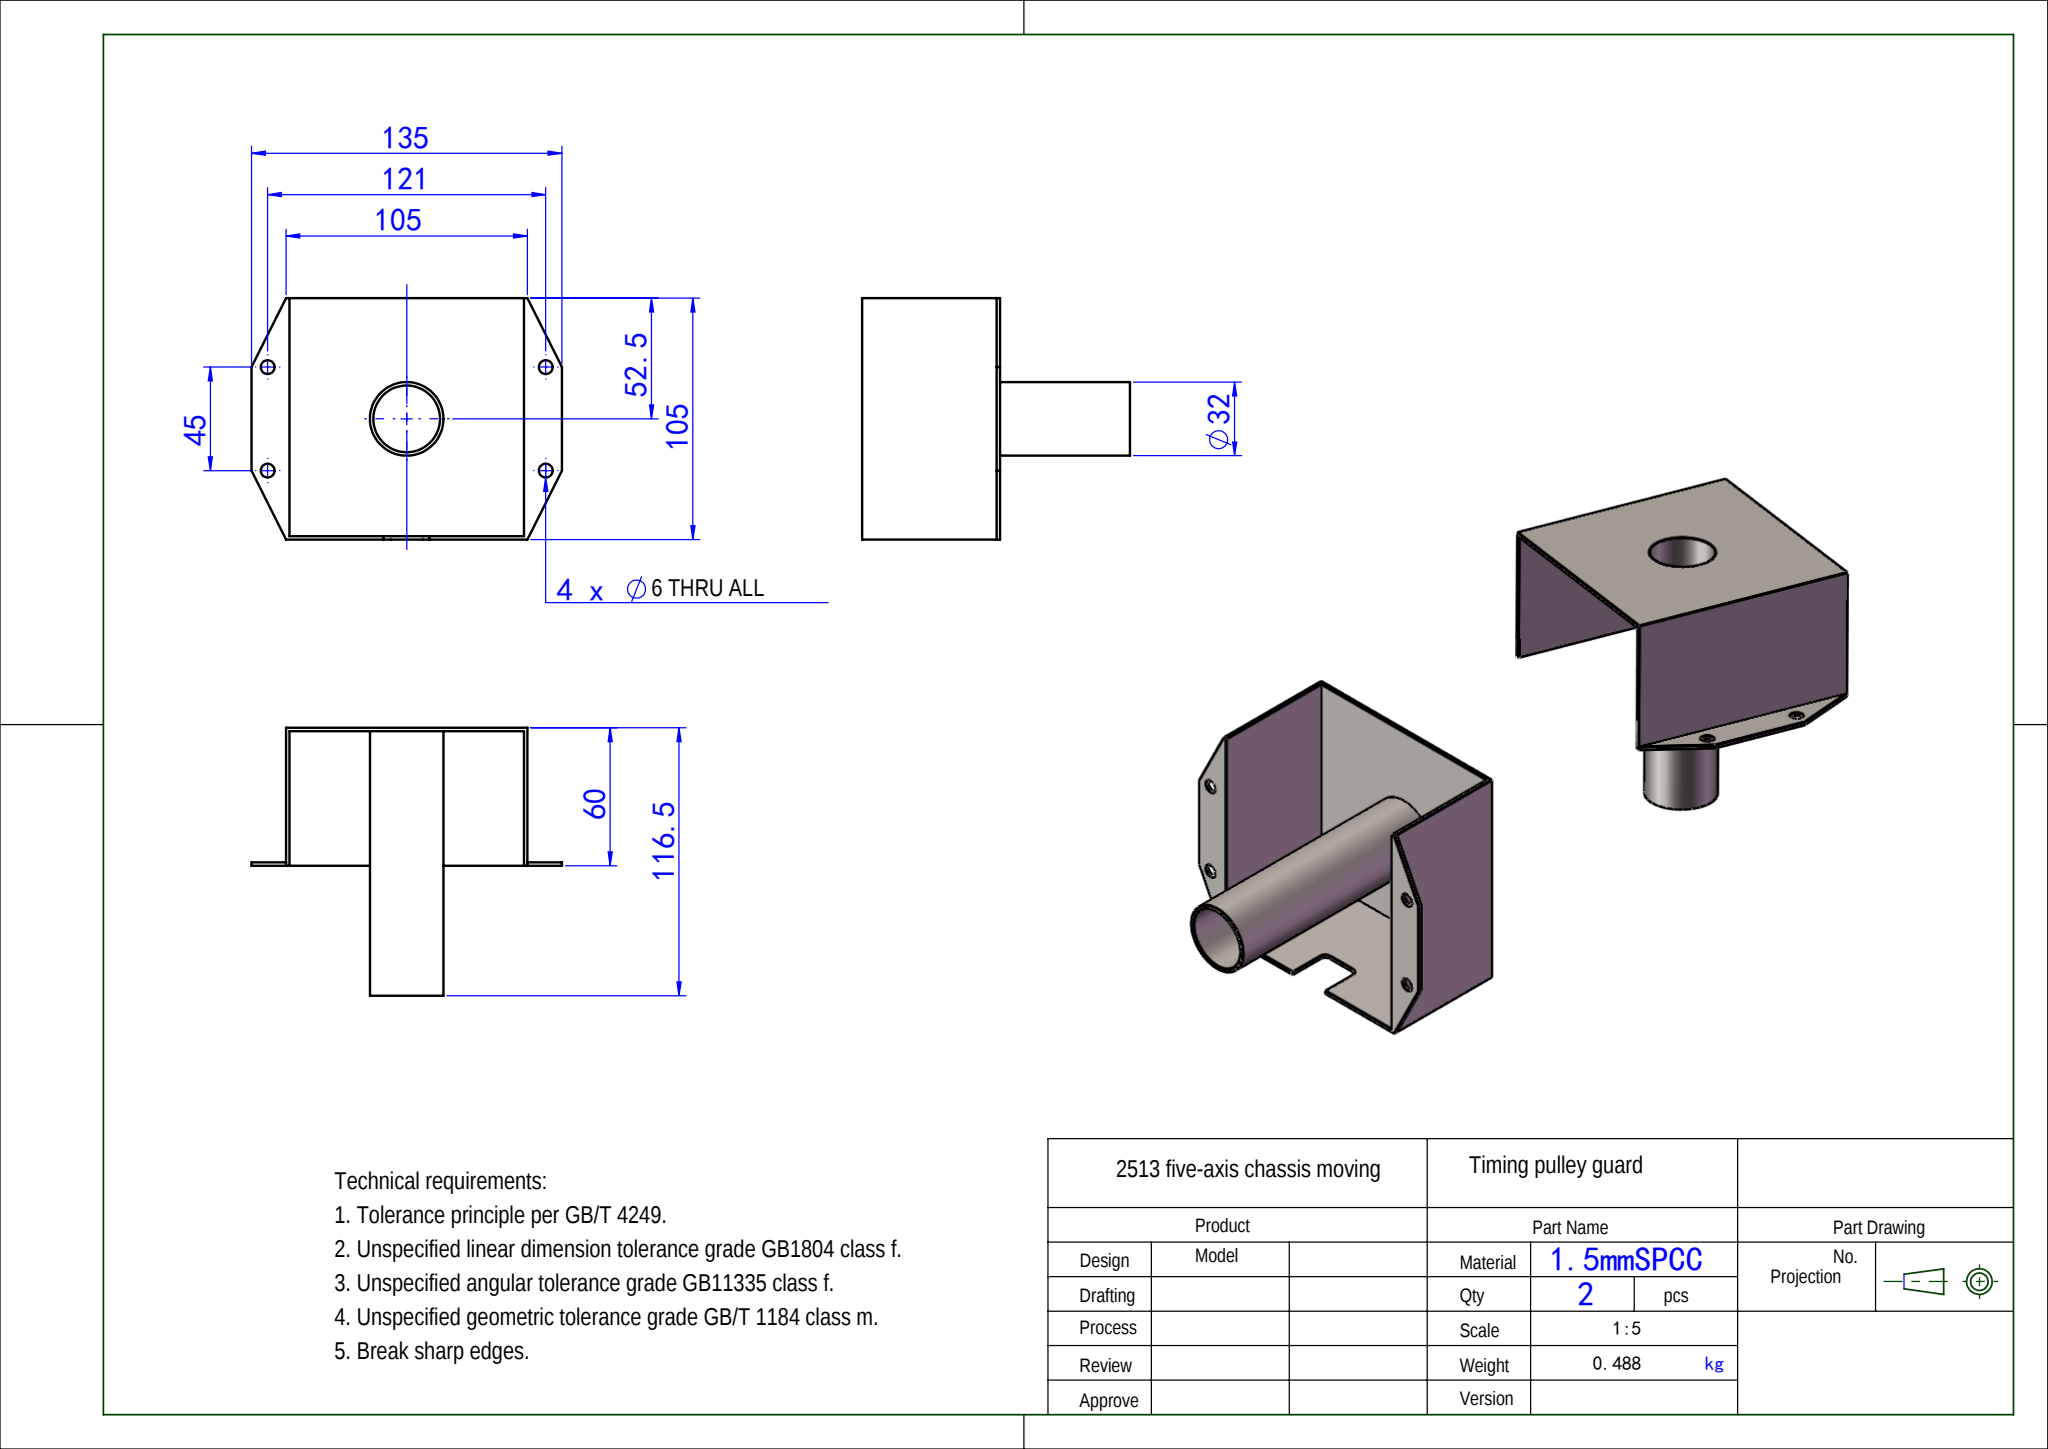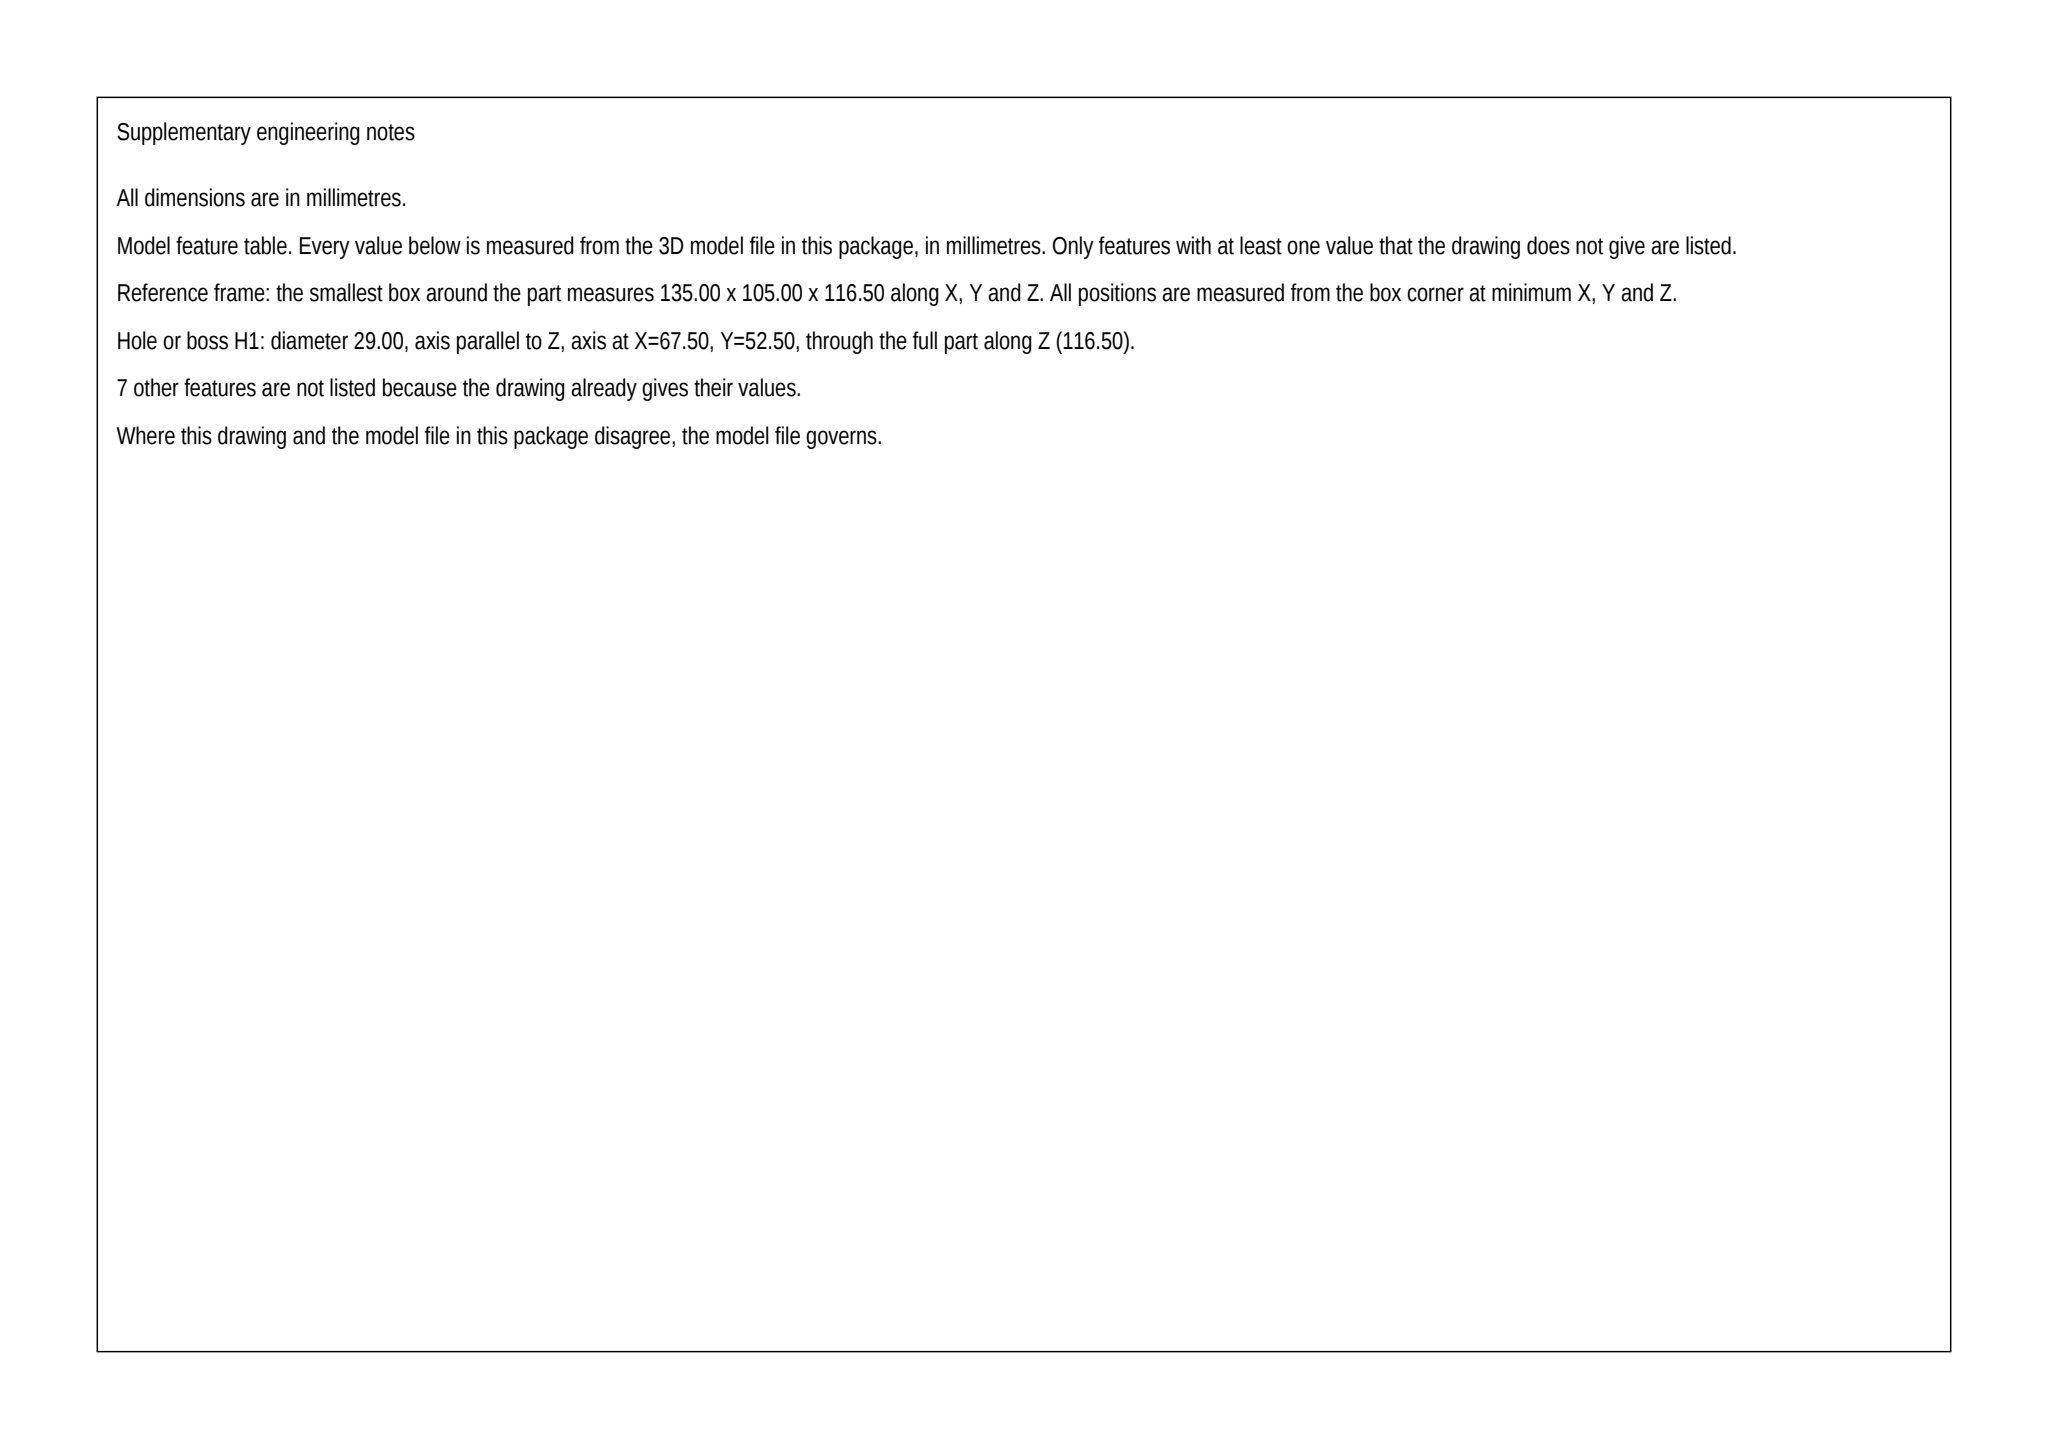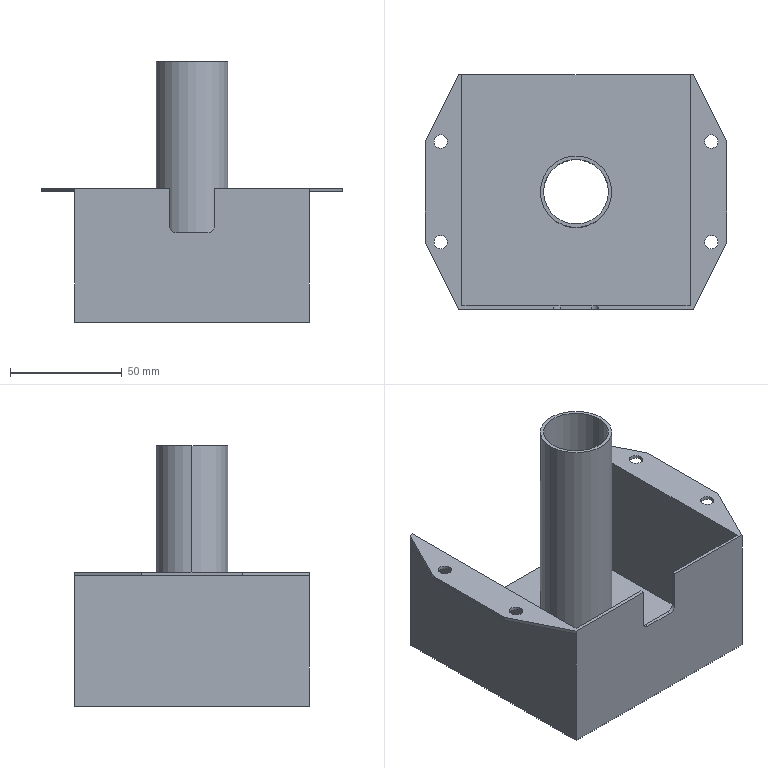Part | SolidWorks | mm | 1 solid | 37 faces | box 135 x 105 x 116.5 mm | volume 62065 mm3 | plane 23 | cylinder 14 | commonest cylinder face diameters 6 x10 29 x2 32 x2
Drawing notes:
4X C15 X 45 ON PLATE CORNERS (135 & 105 EDGES), TYP | from the solid: X-planes 0/135 outer, 135-105=30 -> 15 per side; plane x=15.0; balloon 4 angle 45 deg gives equal legs 15
BTM NOTCH 20 WIDE SYM ABOUT Ø32 CL, 20 DP FROM FLANGE EDGE | from the solid: X-planes 57.5 & 77.5 (20 wide), midpoint 67.5 = Ø32 axis x=67.5; Z-planes 40.0 to 60.0 = 20 deep from flange face z=60